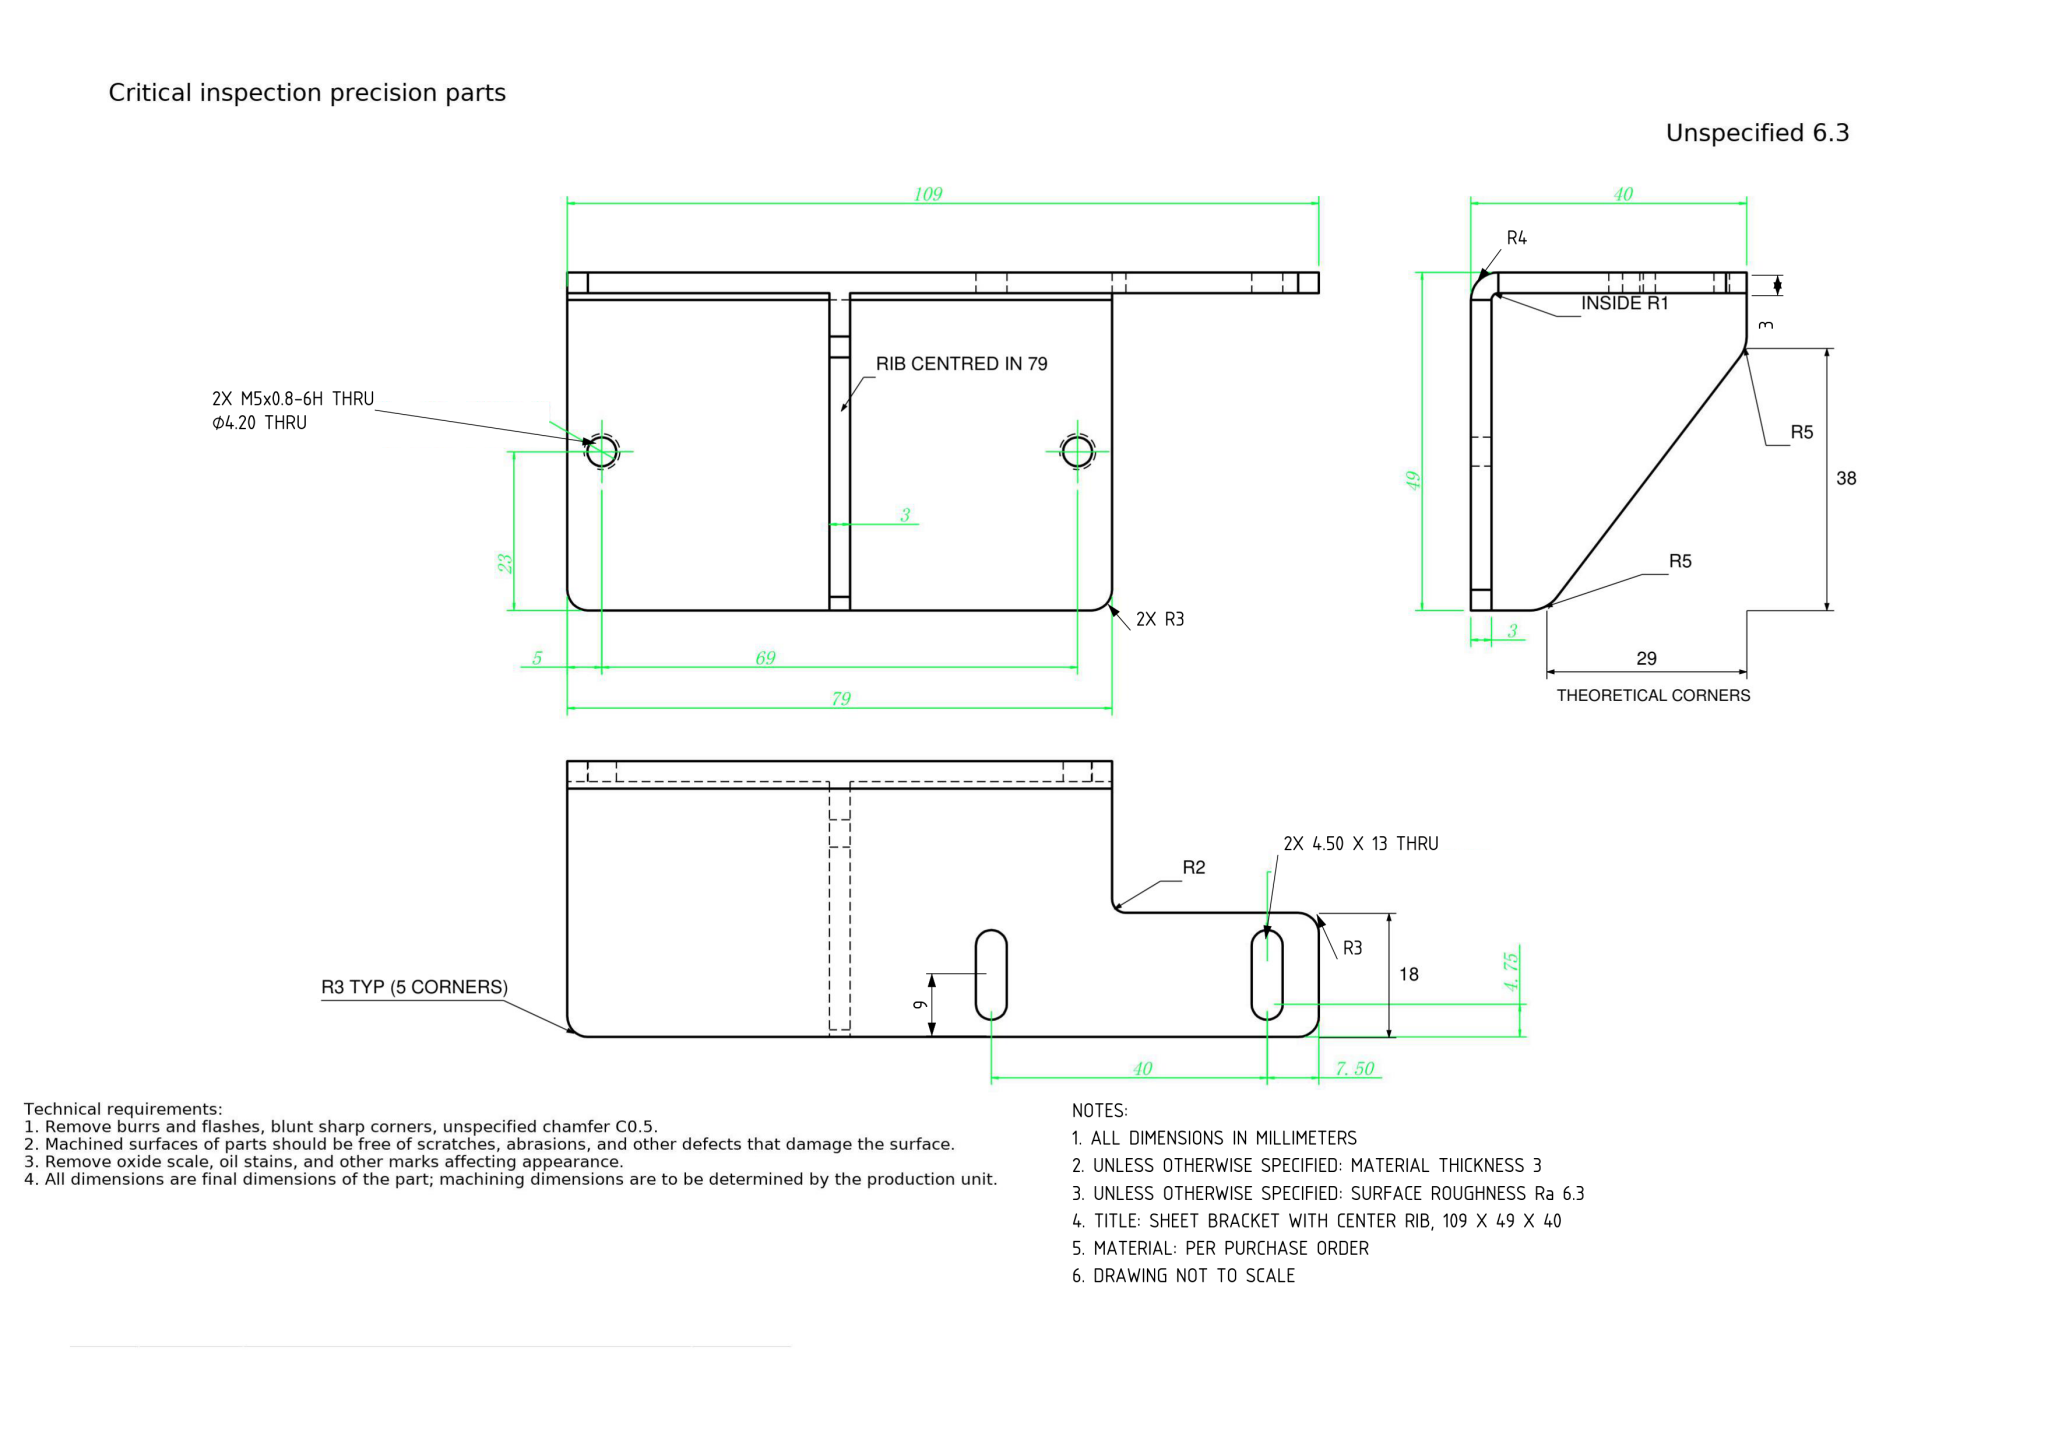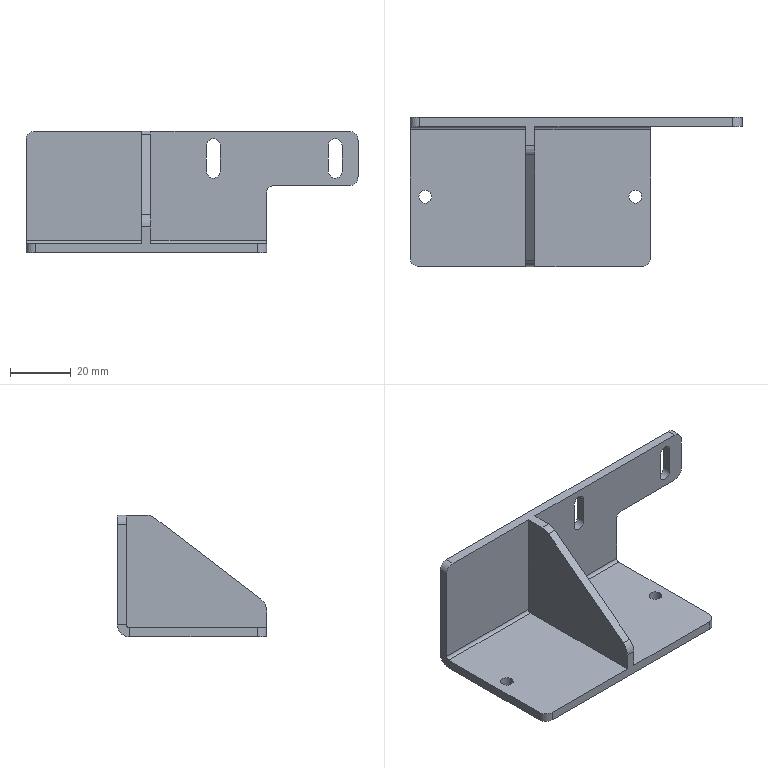Part | NX | mm | 1 solid | 44 faces | box 109 x 49 x 40 mm | volume 24762 mm3 | plane 23 | cylinder 21 | commonest cylinder face diameters 4.5 x6 6 x5 4.2 x4 2 x2 10 x2 8 x1 4 x1